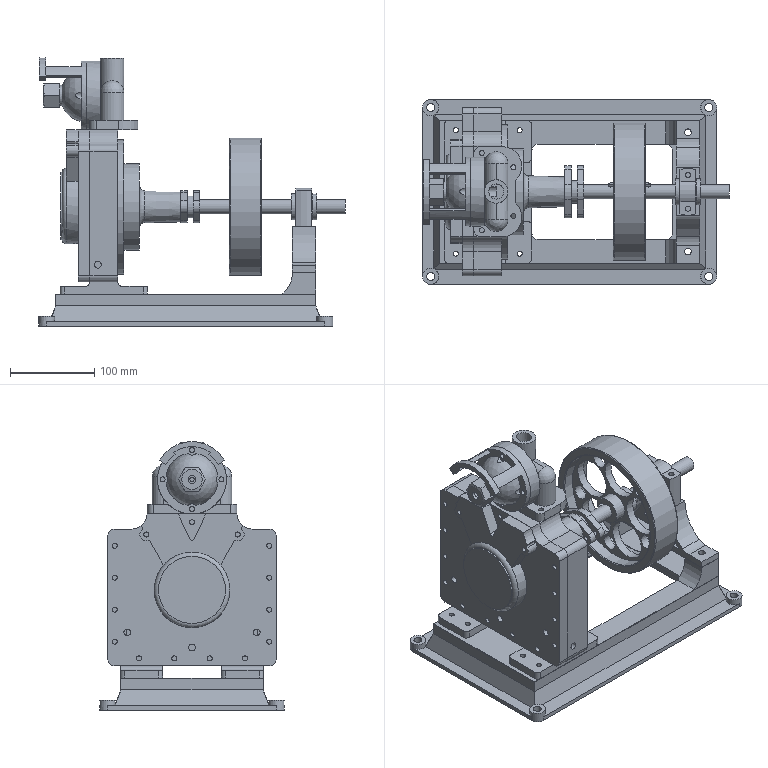Assembly | NX | mm | 33 component files | 33 solids | 786 faces | box 365 x 220 x 319.5 mm | volume 3205377 mm3 | plane 394 | cylinder 377 | torus 8 | sphere 4 | cone 3 | commonest cylinder face diameters 6 x98 5 x41 9 x26 8 x17 10 x16 13 x14 17 x11 15 x10
Bill of materials:
unnamed part 1 | 1 |  | Thick circular disc with four rounded trapezoidal through-cutouts arranged around the center and one small round through-hole near the outer edge.
unnamed part 2 | 1 |  | Bridge-shaped bracket: flat base strip with end flanges, a raised rectangular top pad joined by concave curved flanks, and a trapezoidal window through the raised section.
unnamed part 3 | 1 |  | Plain cylindrical tube/sleeve with uniform wall thickness and open ends.
unnamed part 4 | 1 |  | Rectangular open frame with a stepped (rebated) profile on one face and an obround slot through each short side.
unnamed part 5 | 1 |  | Long rectangular bar with a shallow stepped recess along the middle of one face, leaving raised end sections.
unnamed part 6 | 1 |  | Flat plate with one straight edge and an outline made of two large rounded lobes on the other side, with two obround slots and several round through-holes.
unnamed part 7 | 1 |  | Thick rectangular plate with rounded corners, a large central through-bore, a pattern of small holes on the face, and a raised top tab with concave transitions, notches and small holes.
unnamed part 8 | 1 |  | Long slender stepped cylindrical shaft with a short smaller-diameter end, a short larger collar section, and a long main section with a shallow flat.
unnamed part 9 | 1 |  | Solid plain cylinder (round rod/pin segment) with flat ends.
unnamed part 10 | 1 |  | T-shaped body: obround block with fully rounded ends and edges, with a hollow cylindrical boss rising perpendicular from its top and three through-holes in the block face.
unnamed part 11 | 1 |  | Thick circular disc with two offset round through-holes of different sizes lying along one diameter.
unnamed part 12 | 2 |  | Rectangular plate with rounded corners, a raised central band with concave fillets running across its width, and six round through-holes in two rows of three.
unnamed part 13 | 1 |  | Diamond/oval two-hole flange plate with a cylindrical hub boss projecting from one face and a large central through bore.
unnamed part 14 | 1 |  | Long slender bar of rectangular section that tapers in thickness along its length, with a stepped or sloped transition region on its top face.
unnamed part 15 | 1 |  | Flanged housing: a round flange with four bolt holes and a bowl-shaped recess, a rear domed shell ending in a cylindrical boss, and two parallel arms joining it to a partial-arc ring flange at the far end.
unnamed part 16 | 1 |  | Hexagonal prism with a central cylindrical through bore and a chamfer on one end face (hex-nut-like form).
unnamed part 17 | 1 |  | Wheel- or pulley-like disc with a wide cylindrical rim, a recessed web pierced by five large and five small circular lightening holes, and a central hub bore with a small keyway-like notch.
unnamed part 18 | 1 |  | Flanged cylindrical bushing/sleeve: a short tube with a larger-diameter flange at one end and a through bore.
unnamed part 19 | 1 |  | Flat rectangular plate with rounded corners, two concave radiused notches at the top corners leaving a raised central tab, one large central through hole, and many small holes arranged around the perimeter.
unnamed part 20 | 1 |  | Thick plate shaped as a circular sector (fan) with a tapered tab extending from the narrow end, ending in a rounded tip, and one through hole near the junction.
unnamed part 21 | 1 |  | Elongated bar of square or near-square cross-section with fully rounded ends (parallel-key-like form).
unnamed part 22 | 2 |  | Rectangular block with a concave quarter-round (cove) cut along one edge and a single round through hole perpendicular to the top face.
unnamed part 23 | 2 |  | C-channel (U-section) bracket with a long straight slot with rounded ends through the web.
unnamed part 24 | 1 |  | Flat plate outline made of a circular lower lobe and two diverging upper arms forming a V-notch, with a small eye tab holding a small hole on each arm, and a thin raised circular disc or boss on one face.
unnamed part 25 | 1 |  | Rectangular plate with rounded corners. A raised rectangular platform sits on it, joined by a sloped (chamfer-like) transition. The platform has a rectangular through-cutout with rounded corners and a pattern of small holes. Four corner holes sit on small cylindrical bosses.
unnamed part 26 | 1 |  | Short, thick-walled cylindrical tube (sleeve or spacer-like ring) with a plain coaxial through-bore.
unnamed part 27 | 1 |  | Thin, roughly circular disc with a central through-hole. A thicker rectangular band or block runs across one face, with stepped tabs at its ends where it passes the disc edge. The block has smaller cross-holes and an end slot.
unnamed part 28 | 1 |  | Flanged hub or adapter. A large circular flange carries a raised cylindrical boss and a tapered neck. The neck ends in a small oval two-hole flange with a central bore.
unnamed part 29 | 1 |  | Block-shaped housing with a raised arched middle section and two ears. Each ear has a vertical through-hole. A horizontal through-bore is surrounded by a circular raised collar or boss on its faces. The overall shape resembles a pillow-block-style housing.
unnamed part 30 | 1 |  | Plain cylindrical ring with a fairly thin wall and a large coaxial through-bore. It is shorter axially than unnamed part 26 relative to its diameter.
Mates:
1. fix | base 1 component
2. parallel | spacer_block 2 face | base 1 face
3. parallel | spacer_block 1 face | spacer_block 2 face
4. concentric | spacer_block 2 edge | base 1 arc
5. concentric | spacer_block 1 edge | base 1 arc
6. concentric | base 1 edge | cylinder_body_support_leg 2 edge
7. parallel | cylinder_body_support_leg 2 face | base 1 face
8. concentric | base 1 edge | cylinder_body_support_leg 1 edge
9. parallel | cylinder_body_support_leg 1 face | base 1 face
10. touch align | cylinder_body_support_leg 1 face | cylinder_body 1 face
11. center | cylinder_body 1 face | cylinder_body 1 face | cylinder_body_support_leg 2 face | cylinder_body_support_leg 1 face
12. center | cylinder_body 1 face | cylinder_body 1 face | cylinder_body_support_leg 1 face | cylinder_body_support_leg 1 face
13. concentric | rear_cylinder_head 1 edge | cylinder_body 1 edge
14. concentric | rear_cylinder_head 1 edge | cylinder_body 1 edge
15. concentric | long_bushing 1 arc | rear_cylinder_head 1 edge
16. concentric | short_bushing 1 arc | long_bushing 1 edge
17. concentric | outer_end_cap 1 edge | short_bushing 1 edge
18. touch align | outer_end_cap 1 face | rear_cylinder_head 1 face
19. concentric | cylinder_body 1 edge | front_end_cap 1 arc
20. parallel | front_end_cap 1 face | cylinder_body 1 face
21. concentric | front_end_cap 1 edge | front_outer_end_cap 1 arc
22. parallel | front_outer_end_cap 1 face | front_end_cap 1 face
23. touch align | lower_wedge 1 face | cylinder_body 1 face
24. touch align | cylinder_body 1 face | lower_wedge 1 face
25. touch align | cylinder_body 1 face | lower_wedge 1 edge
26. touch align | upper_wedge 1 face | lower_wedge 1 face
27. touch align | upper_wedge 1 edge | cylinder_body 1 face
28. touch align | frame 1 face | cylinder_body 1 face
29. touch align | frame 1 face | cylinder_body 1 face
30. touch align | side_support_frame 2 | frame 1 face
31. touch align | cylinder_body 1 face | side_support_frame 2
32. touch align | side_support_frame 1 face | frame 1 face
33. touch align | side_support_frame 1 face | cylinder_body 1 face
34. concentric | cylinder_body 1 edge | upper_top_plate 1 arc
35. parallel | upper_top_plate 1 face | front_end_cap 1 face
36. concentric | upper_cylinder_body 1 arc | upper_top_plate 1 edge
37. parallel | upper_cylinder_body 1 face | upper_top_plate 1 face
38. concentric | upper_top_plate 1 edge | outer_support_plate 1 arc
39. parallel | outer_support_plate 1 face | upper_top_plate 1 face
40. concentric | outer_support_plate 1 edge | front_mount_end_cap 1 edge
41. concentric | front_mount_end_cap 1 arc | outer_support_plate 1 edge
42. concentric | washer 1 arc | front_mount_end_cap 1 edge
43. concentric | bushing 1 | washer 1
44. concentric | large_nut 1 | bushing 1 arc